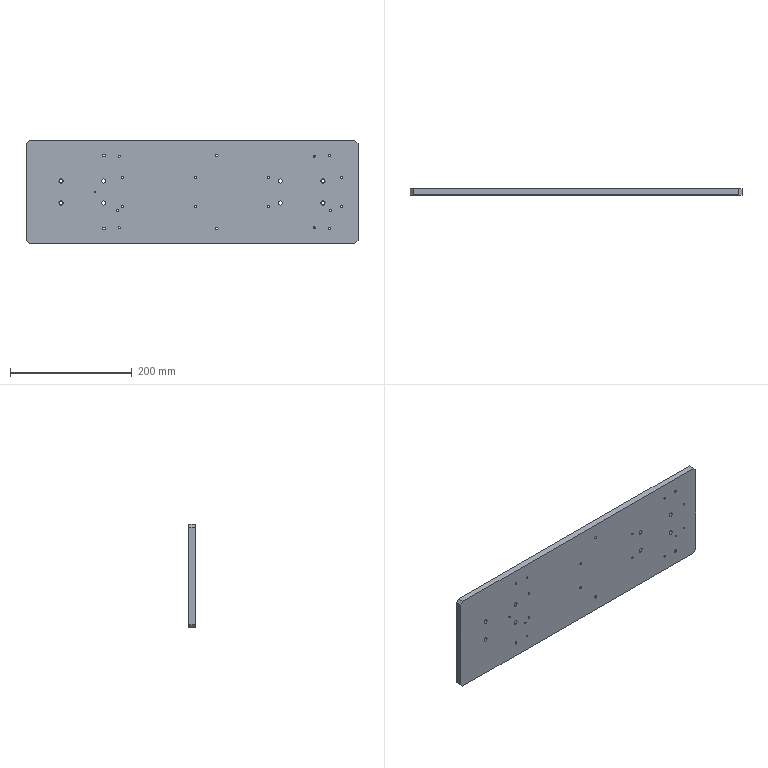Component | SolidWorks | SFTJ-03-XModuleBackPlate-1 | 1 solid | 80 faces | box 545 x 10 x 170 mm | volume 920817 mm3 | cylinder 64 | plane 10 | cone 6 | commonest cylinder face diameters 3.3 x22 6.8 x16 3 x14 4.2 x12 | material 45
build123d program:
from build123d import *

# Parameters (mm, degrees)
SKETCH1_W                   = 545
SKETCH1_H                   = 170
BOSS_EXTRUDE1_DEPTH         = 5
CHAMFER1_SIZE               = 5
SIZE_MM_DOWEL_PIN_HOLE0_D   = 3
M4_TAPPED_HOLE1_D           = 3.3
SIZE_MM_DOWEL_PIN_HOLE1_D   = 3
M8_TAPPED_HOLE1_D           = 6.8
M5_TAPPED_HOLE1_D           = 4.2
M5_TAPPED_HOLE2_D           = 4.2
M4_TAPPED_HOLE2_D           = 3.3
M4_TAPPED_HOLE2_DEPTH       = 10.1
M4_TAPPED_HOLE2_TIP         = 0.9914
SIZE_MM_DOWEL_PIN_HOLE0_2_D = 3


with BuildPart() as part:
    # Sketch1 → Boss-Extrude1 (new, symmetric)
    with BuildSketch(Plane.XY):
        Rectangle(SKETCH1_W, SKETCH1_H)
    extrude(amount=BOSS_EXTRUDE1_DEPTH, both=True)

    # Chamfer1
    chamfer1_edges = [part.edges().sort_by_distance(p)[0] for p in [
        (272.5, -85, 0),
        (-272.5, -85, 0),
        (-272.5, 85, 0),
        (272.5, 85, 0),
    ]]
    chamfer(chamfer1_edges, length=CHAMFER1_SIZE)

    # Size mm Dowel Pin Hole0 (through all)
    with Locations(Plane(origin=(0, 0, -5), x_dir=(-1, 0, 0), z_dir=(0, 0, -1))):
        with Locations((122.5, -30.5), (-227.5, -30.5)):
            Hole(SIZE_MM_DOWEL_PIN_HOLE0_D / 2)

    # M4 Tapped Hole1 (through all)
    with Locations(Plane(origin=(0, 0, -5), x_dir=(-1, 0, 0), z_dir=(0, 0, -1))):
        with Locations((114.25, -24), (114.25, 24), (-5.75, 24), (-5.75, -24), (-125.75, -24), (-125.75, 24), (-245.75, -24), (-245.75, 24)):
            Hole(M4_TAPPED_HOLE1_D / 2)

    # Size mm Dowel Pin Hole1 (through all)
    with Locations(Plane(origin=(0, 0, -5), x_dir=(-1, 0, 0), z_dir=(0, 0, -1))):
        with Locations((159.25, 0)):
            Hole(SIZE_MM_DOWEL_PIN_HOLE1_D / 2)

    # M8 Tapped Hole1 (through all)
    with Locations(Plane.XY.offset(5)):
        with Locations((215, -18), (215, 18), (145, -18), (145, 18), (-145, -18), (-145, 18), (-215, -18), (-215, 18)):
            Hole(M8_TAPPED_HOLE1_D / 2)

    # M5 Tapped Hole1 (through all)
    with Locations(Plane(origin=(0, 0, -5), x_dir=(-1, 0, 0), z_dir=(0, 0, -1))):
        with Locations((144.25, -60), (-40.75, -60), (-225.75, -60)):
            Hole(M5_TAPPED_HOLE1_D / 2)

    # M5 Tapped Hole2 (through all)
    with Locations(Plane(origin=(0, 0, -5), x_dir=(-1, 0, 0), z_dir=(0, 0, -1))):
        with Locations((144.25, 60), (-40.75, 60), (-225.75, 60)):
            Hole(M5_TAPPED_HOLE2_D / 2)

    # M4 Tapped Hole2
    with Locations(Plane(origin=(0, -85, 0), x_dir=(-1, 0, 0), z_dir=(0, -1, 0))):
        with Locations((-235.75, 0), (-110.75, 0), (14.25, 0)):
            Hole(M4_TAPPED_HOLE2_D / 2, depth=M4_TAPPED_HOLE2_DEPTH)
            with Locations((0, 0, -(M4_TAPPED_HOLE2_DEPTH + M4_TAPPED_HOLE2_TIP / 2))):  # 118° drill point
                Cone(0, M4_TAPPED_HOLE2_D / 2, M4_TAPPED_HOLE2_TIP, mode=Mode.SUBTRACT)

    # Size mm Dowel Pin Hole0_2 (through all)
    with Locations(Plane(origin=(0, 0, -5), x_dir=(-1, 0, 0), z_dir=(0, 0, -1))):
        with Locations((119.25, 58.5), (-200.75, -58.5), (119.25, -58.5), (-200.75, 58.5)):
            Hole(SIZE_MM_DOWEL_PIN_HOLE0_2_D / 2)


solid = part.part

# Placed as in the assembly
solid = solid.moved(Location((-137.759, -12.279, 38.589), (90, 0, 0)))